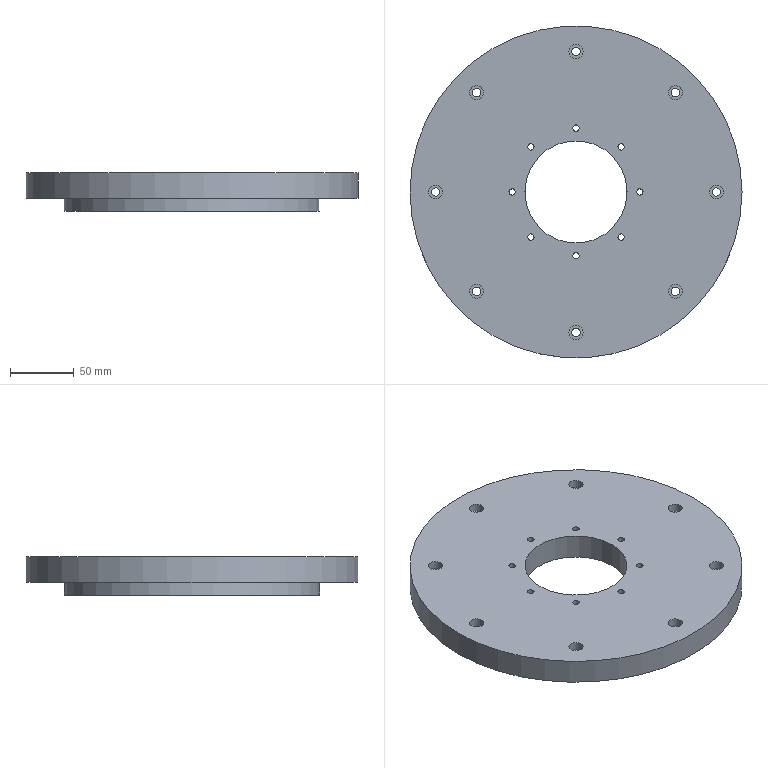Component | NX | SENSOR_PLATE | 1 solid | 40 faces | volume 1009093 mm3 | cylinder 28 | plane 12 | commonest cylinder face diameters 6.6 x8 11 x8 5 x8 260 x1 200 x1 180 x1 80 x1